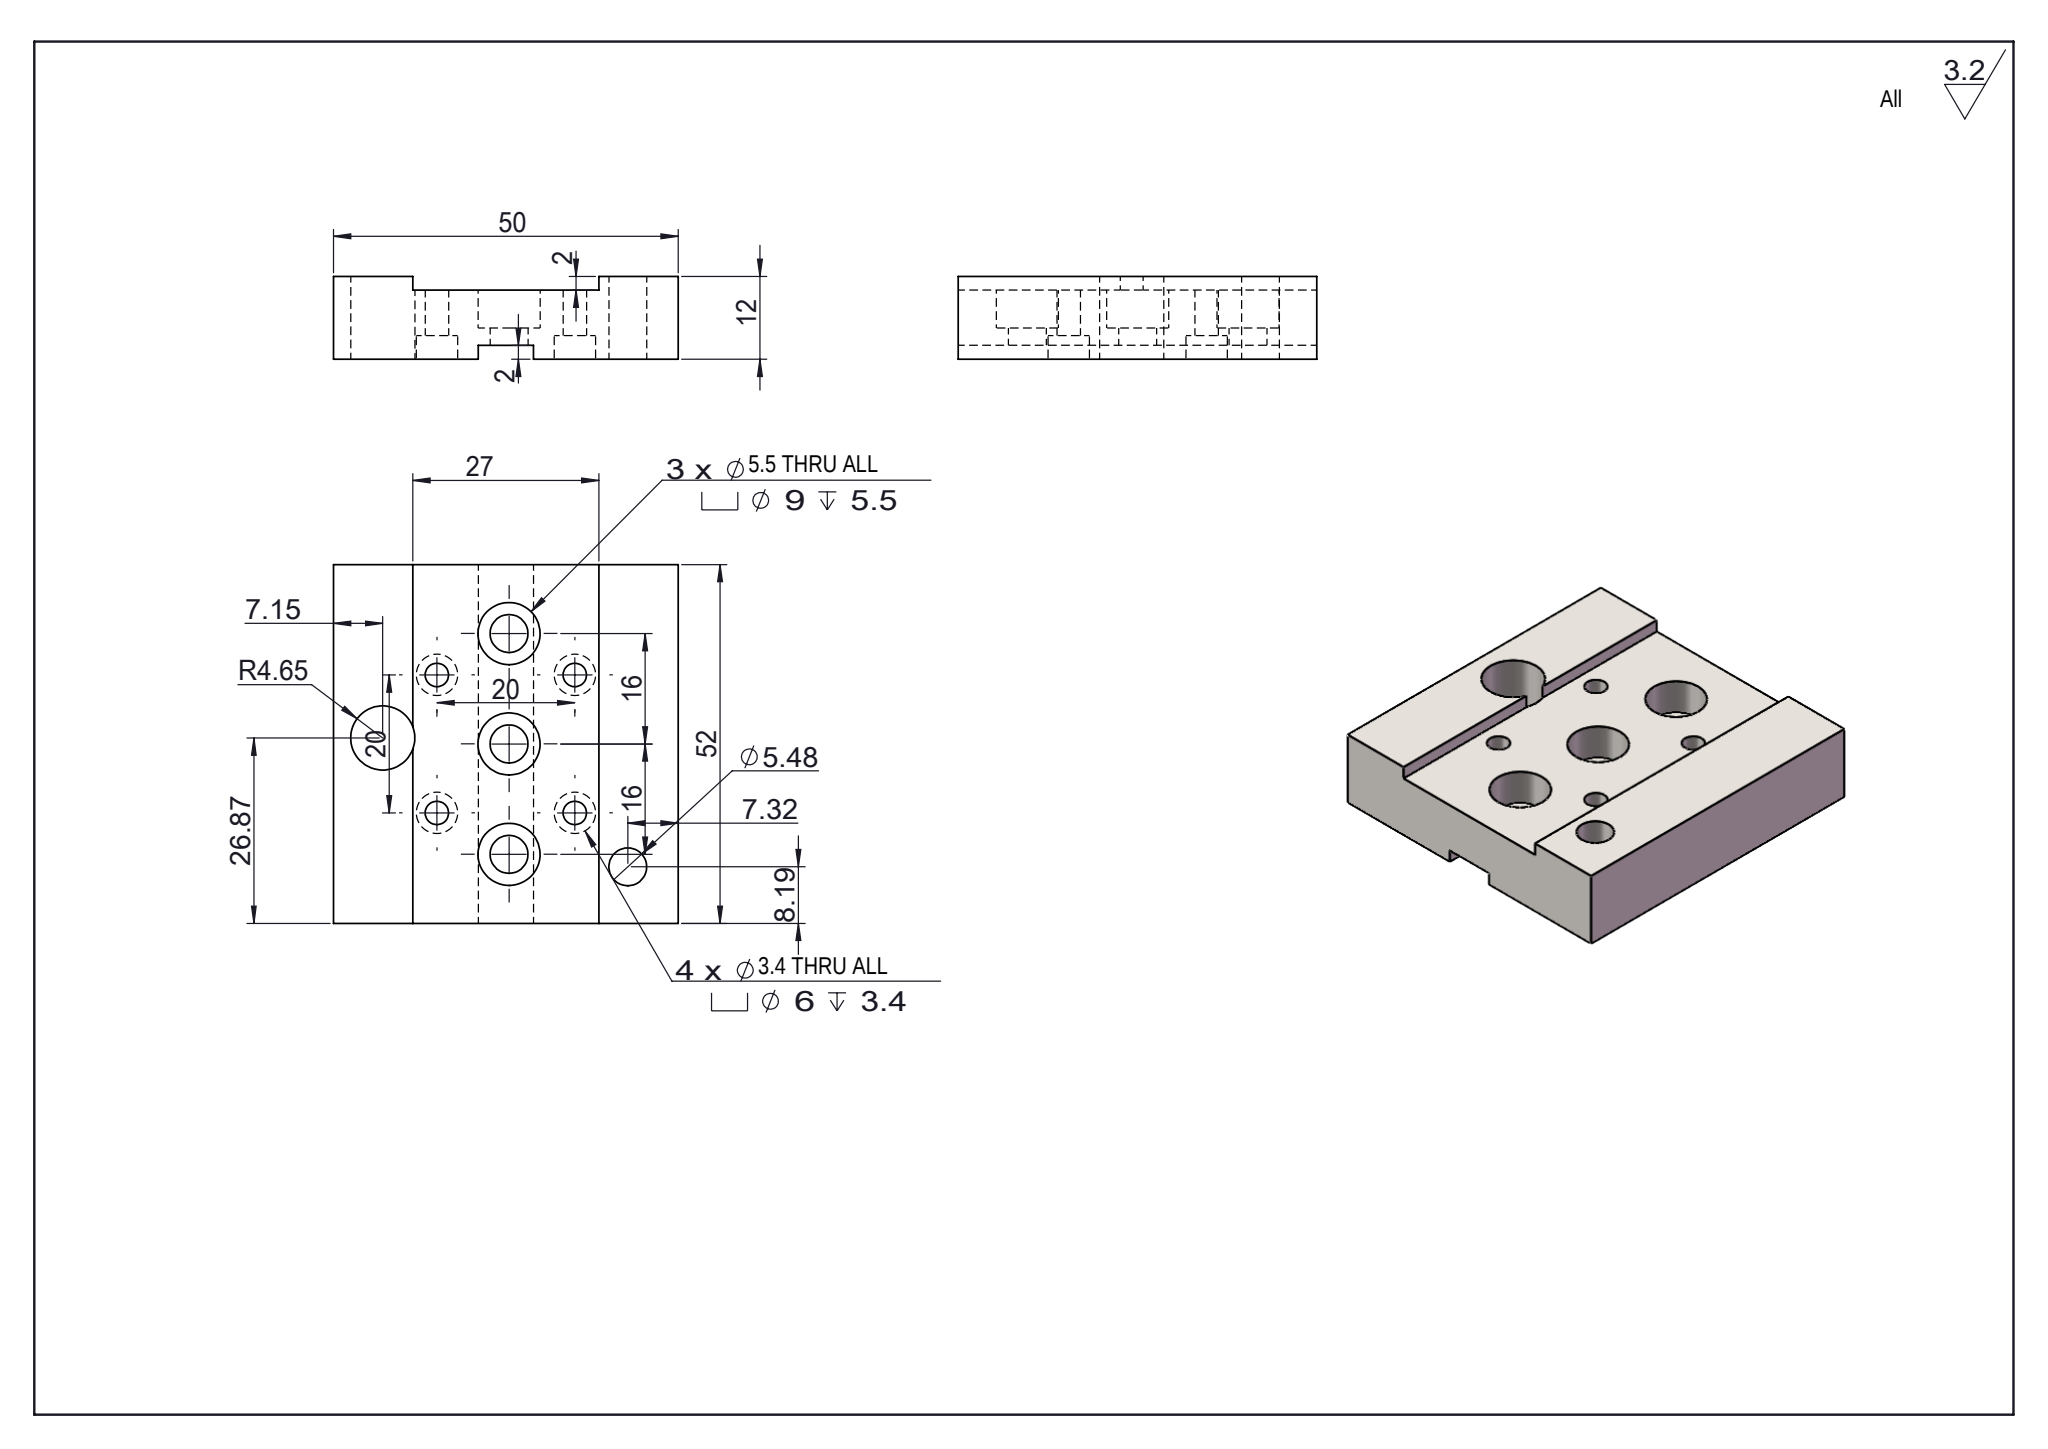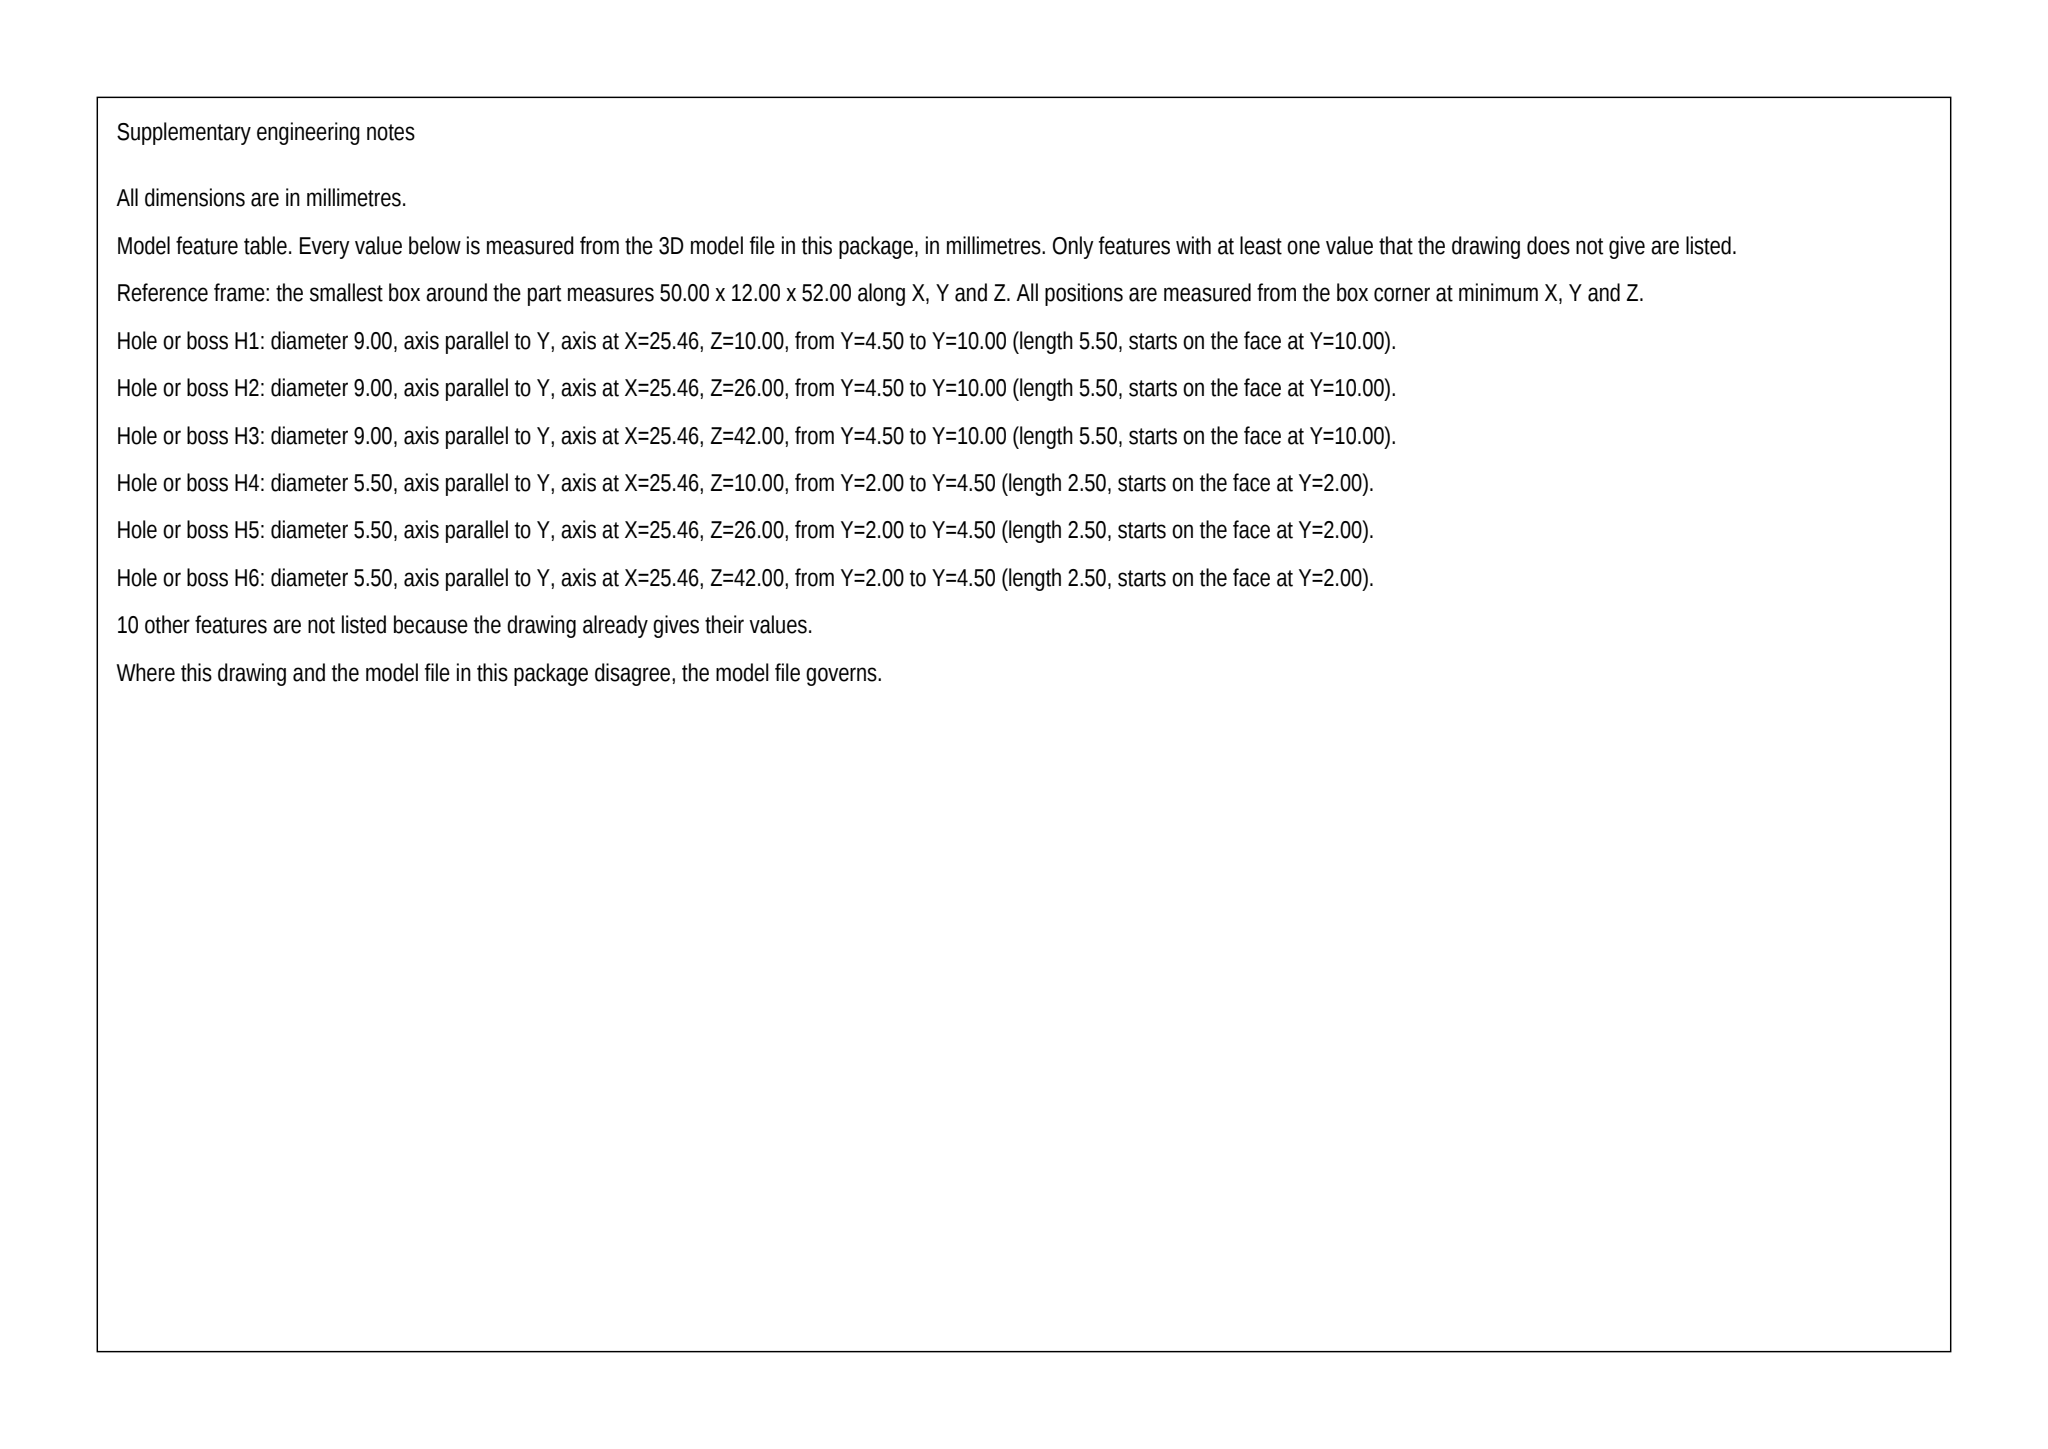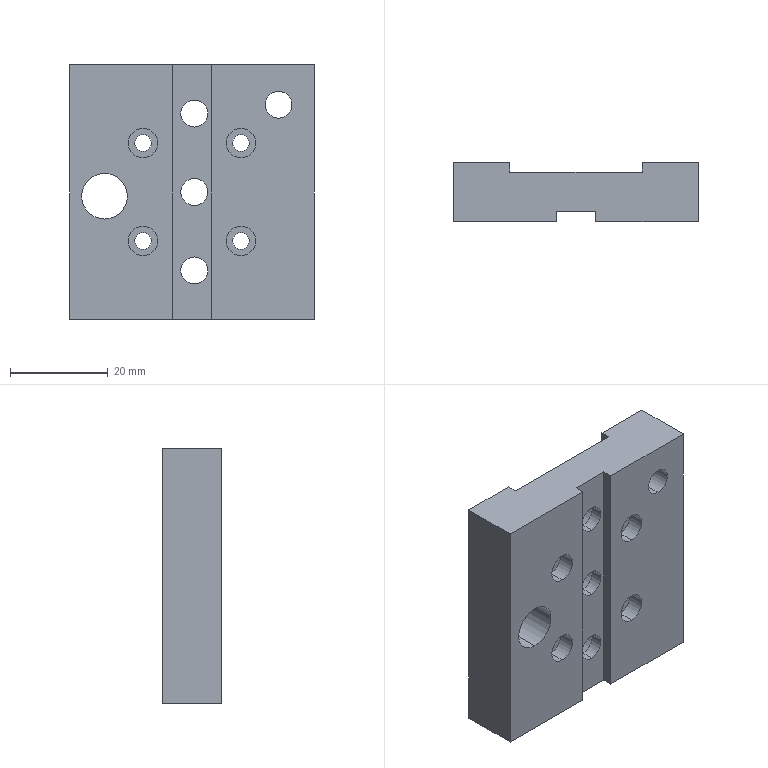Part | SolidWorks | mm | 1 solid | 54 faces | box 50 x 12 x 52 mm | volume 24610 mm3 | cylinder 32 | plane 22 | commonest cylinder face diameters 6 x8 3.4 x8 9 x6 5.5 x6 5.479 x2 9.305 x2
build123d program:
from build123d import *

# Parameters (mm, degrees)
BOSS_EXTRUDE1_DEPTH                                  = 52
SKETCH2_W                                            = 27
SKETCH2_H                                            = 52
CUT_EXTRUDE1_DEPTH                                   = 2
CYLINDRICAL_COUNTERSUNK_HOLE_1_FOR_M5_HE_D           = 5.5
CYLINDRICAL_COUNTERSUNK_HOLE_1_FOR_M5_HE_CBORE_D     = 9
CYLINDRICAL_COUNTERSUNK_HOLE_1_FOR_M5_HE_CBORE_DEPTH = 5.5
CYLINDRICAL_COUNTERSUNK_HOLE_1_FOR_M3_HE_D           = 3.4
CYLINDRICAL_COUNTERSUNK_HOLE_1_FOR_M3_HE_CBORE_D     = 6
CYLINDRICAL_COUNTERSUNK_HOLE_1_FOR_M3_HE_CBORE_DEPTH = 3.4
SKETCH7_R                                            = 2.739
SKETCH7_R_2                                          = 4.652
CUT_EXTRUDE2_DEPTH                                   = 80


with BuildPart() as part:
    # Sketch1 → Boss-Extrude1 (new body)
    with BuildSketch(Plane.XY):
        Polygon((0, 28), (0, 30), (8, 30), (8, 28), (29, 28), (29, 40), (-21, 40), (-21, 28), align=None)
    extrude(amount=-BOSS_EXTRUDE1_DEPTH)

    # Sketch2 → Cut-Extrude1 (cut)
    with BuildSketch(Plane(origin=(0, 40, 0), x_dir=(1, 0, 0), z_dir=(0, 1, 0))):
        with Locations((4, 26)):
            Rectangle(SKETCH2_W, SKETCH2_H)
    extrude(amount=-CUT_EXTRUDE1_DEPTH, mode=Mode.SUBTRACT)

    # Cylindrical Countersunk Hole 1 for M5 He (through all)
    with Locations(Plane(origin=(0, 38, 0), x_dir=(1, 0, 0), z_dir=(0, 1, 0))):
        with Locations((4.465, 42), (4.465, 26), (4.465, 10)):
            CounterBoreHole(CYLINDRICAL_COUNTERSUNK_HOLE_1_FOR_M5_HE_D / 2, CYLINDRICAL_COUNTERSUNK_HOLE_1_FOR_M5_HE_CBORE_D / 2, CYLINDRICAL_COUNTERSUNK_HOLE_1_FOR_M5_HE_CBORE_DEPTH)

    # Cylindrical Countersunk Hole 1 for M3 He (through all)
    with Locations(Plane(origin=(0, 28, 0), x_dir=(-1, 0, 0), z_dir=(0, -1, 0))):
        with Locations((-14, 16), (6, 16), (-14, 36), (6, 36)):
            CounterBoreHole(CYLINDRICAL_COUNTERSUNK_HOLE_1_FOR_M3_HE_D / 2, CYLINDRICAL_COUNTERSUNK_HOLE_1_FOR_M3_HE_CBORE_D / 2, CYLINDRICAL_COUNTERSUNK_HOLE_1_FOR_M3_HE_CBORE_DEPTH)

    # Sketch7 → Cut-Extrude2 (cut)
    with BuildSketch(Plane(origin=(0, 28, 0), x_dir=(-1, 0, 0), z_dir=(0, -1, 0))):
        with Locations(Location((-21.682, 8.19, 0), (0, 0, 90))):
            Circle(SKETCH7_R)
        with Locations(Location((13.848, 26.868, 0), (0, 0, 90))):
            Circle(SKETCH7_R_2)
    extrude(amount=-CUT_EXTRUDE2_DEPTH, mode=Mode.SUBTRACT)


solid = part.part